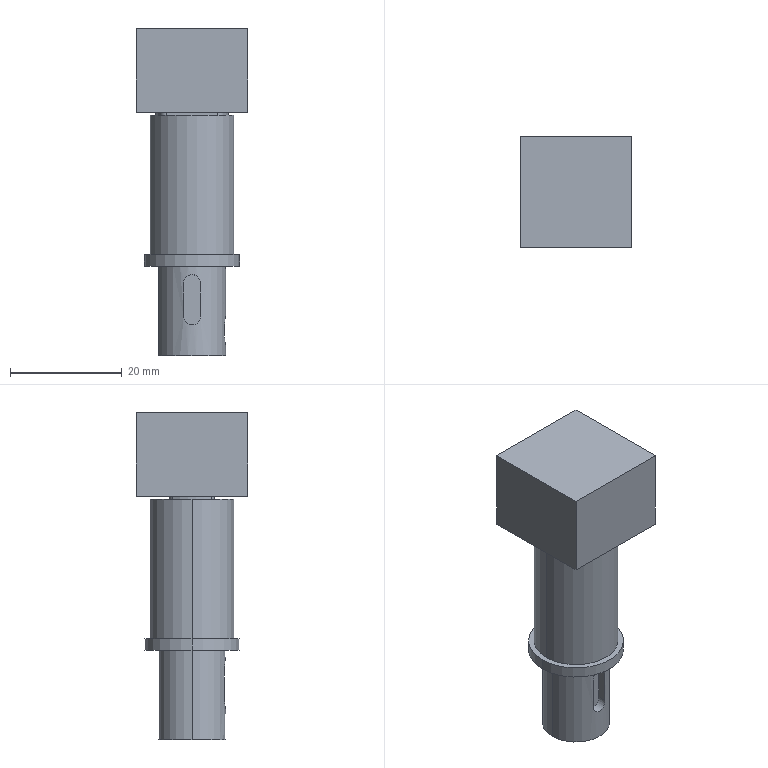CAM job | Mastercam | mm | 17 operations | part box 20 x 20 x 58.5
1. Contour (2D) | 12 - 10 平铣刀
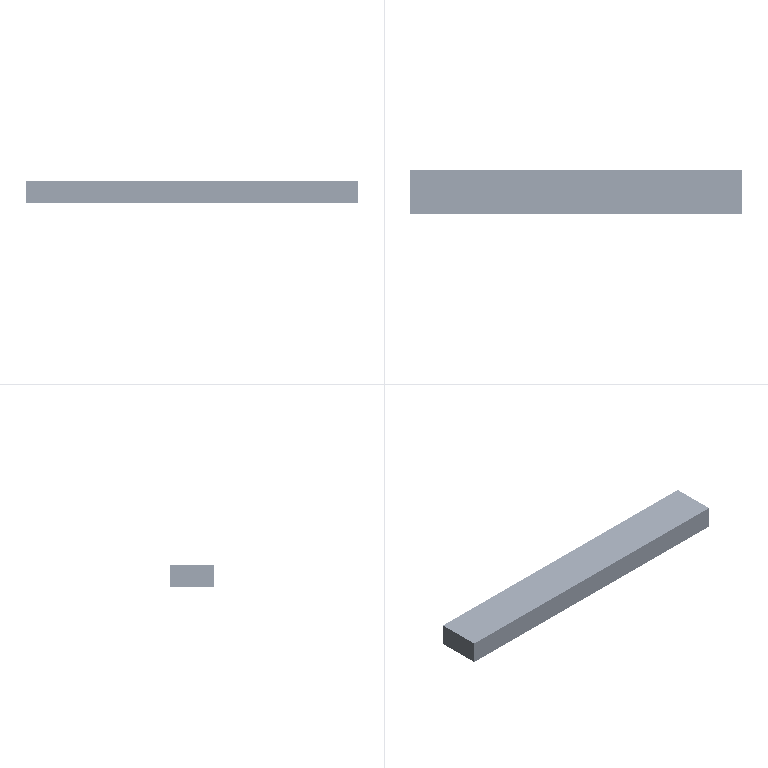2. Contour (2D) | 10 - 12 平铣刀
3. Contour (2D) | 10 - 12 平铣刀
4. Contour (2D chamfer) | 5 - 4 倒角刀
5. Facing | 20 - 63 平铣刀
6. Contour (Ramp) | 8 - 8 平铣刀
7. Contour (Ramp) | 8 - 8 平铣刀
8. Contour (Ramp) | 4 - 4 平铣刀
9. Contour (Remachining) | 2 - 2 平铣刀
10. Contour (Ramp) | 2 - 2 平铣刀
11. 2D High Speed (2D Area Mill) | 2 - 2 平铣刀
12. Contour (2D chamfer) | 5 - 4 倒角刀
13. Contour (Ramp) | 2 - 2 平铣刀
14. Contour (Ramp) | 2 - 2 平铣刀
15. Contour (Ramp) | 15 - 6 平铣刀
16. Contour (2D) | 6 - 6 平铣刀
17. Contour (2D chamfer) | 5 - 4 倒角刀